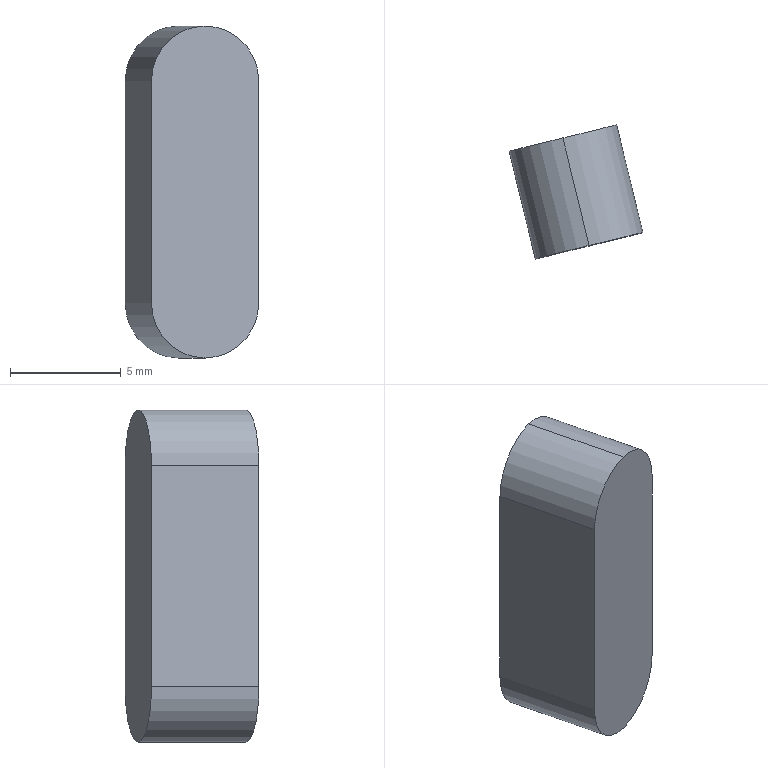Component | SolidWorks | CarrierB5-L15-1 | 1 solid | 7 faces | box 6.04 x 6.04 x 15 mm | volume 348 mm3 | plane 4 | cylinder 3 | commonest cylinder face diameters 5 x3
build123d program:
from build123d import *

# Parameters (mm, degrees)
BOSS_EXTRUDE1_DEPTH = 5


with BuildPart() as part:
    # Sketch1 → Boss-Extrude1 (new body)
    with BuildSketch(Plane(origin=(0, 0, 0), x_dir=(-1, 0, 0), z_dir=(0, 0, -1))):
        with BuildLine():
            Line((-7.5, -2.5), (2.5, -2.5))
            ThreePointArc((2.5, -2.5), (5, 0), (2.5, 2.5))
            Line((2.5, 2.5), (-7.5, 2.5))
            ThreePointArc((-7.5, 2.5), (-10, 0), (-7.5, -2.5))
        make_face()
    extrude(amount=-BOSS_EXTRUDE1_DEPTH)


solid = part.part

# Placed as in the assembly
solid = solid.moved(Location((-20.365, -8.743, 44.5), (-90, -13.725, 90)))
STEP:
#1=COLOUR_RGB('',0.7922,0.8196,0.9333);
#2=FILL_AREA_STYLE_COLOUR('',#1);
#3=FILL_AREA_STYLE('',(#2));
#4=SURFACE_STYLE_FILL_AREA(#3);
#5=SURFACE_SIDE_STYLE('',(#4));
#6=SURFACE_STYLE_USAGE(.BOTH.,#5);
#7=PRESENTATION_STYLE_ASSIGNMENT((#6));
#8=CARTESIAN_POINT('',(-0.7528,-0.1296,1.85));
#9=VERTEX_POINT('',#8);
#10=CARTESIAN_POINT('',(-0.8485,-0.153,1.949));
#11=VERTEX_POINT('',#10);
#12=CARTESIAN_POINT('',(-0.8485,-0.153,1.85));
#13=DIRECTION('',(0.2373,-0.9714,0.));
#14=DIRECTION('',(0.,0.,1.));
#15=AXIS2_PLACEMENT_3D('',#12,#13,#14);
#16=CIRCLE('',#15,0.09843);
#17=EDGE_CURVE('',#9,#11,#16,.T.);
#18=ORIENTED_EDGE('',*,*,#17,.T.);
#19=CARTESIAN_POINT('',(-0.8018,-0.3442,1.949));
#20=VERTEX_POINT('',#19);
#21=CARTESIAN_POINT('',(-0.8485,-0.153,1.949));
#22=DIRECTION('',(0.2373,-0.9714,0.));
#23=VECTOR('',#22,39.37);
#24=LINE('',#21,#23);
#25=EDGE_CURVE('',#11,#20,#24,.T.);
#26=ORIENTED_EDGE('',*,*,#25,.T.);
#27=CARTESIAN_POINT('',(-0.7061,-0.3209,1.85));
#28=VERTEX_POINT('',#27);
#29=CARTESIAN_POINT('',(-0.8018,-0.3442,1.85));
#30=DIRECTION('',(0.2373,-0.9714,0.));
#31=DIRECTION('',(0.,0.,1.));
#32=AXIS2_PLACEMENT_3D('',#29,#30,#31);
#33=CIRCLE('',#32,0.09843);
#34=EDGE_CURVE('',#28,#20,#33,.T.);
#35=ORIENTED_EDGE('',*,*,#34,.F.);
#36=CARTESIAN_POINT('',(-0.7528,-0.1296,1.85));
#37=DIRECTION('',(0.2373,-0.9714,0.));
#38=VECTOR('',#37,39.37);
#39=LINE('',#36,#38);
#40=EDGE_CURVE('',#9,#28,#39,.T.);
#41=ORIENTED_EDGE('',*,*,#40,.F.);
#42=EDGE_LOOP('',(#18,#26,#35,#41));
#43=FACE_OUTER_BOUND('',#42,.T.);
#44=CARTESIAN_POINT('',(-0.8485,-0.153,1.85));
#45=DIRECTION('',(0.2373,-0.9714,0.));
#46=DIRECTION('',(0.,0.,1.));
#47=AXIS2_PLACEMENT_3D('',#44,#45,#46);
#48=CYLINDRICAL_SURFACE('',#47,0.09843);
#49=ADVANCED_FACE('',(#43),#48,.T.);
#50=CARTESIAN_POINT('',(-0.8974,-0.3676,1.457));
#51=VERTEX_POINT('',#50);
#52=CARTESIAN_POINT('',(-0.7061,-0.3209,1.457));
#53=VERTEX_POINT('',#52);
#54=CARTESIAN_POINT('',(-0.8018,-0.3442,1.457));
#55=DIRECTION('',(0.2373,-0.9714,0.));
#56=DIRECTION('',(0.,0.,1.));
#57=AXIS2_PLACEMENT_3D('',#54,#55,#56);
#58=CIRCLE('',#57,0.09843);
#59=EDGE_CURVE('',#51,#53,#58,.T.);
#60=ORIENTED_EDGE('',*,*,#59,.F.);
#61=CARTESIAN_POINT('',(-0.9441,-0.1763,1.457));
#62=VERTEX_POINT('',#61);
#63=CARTESIAN_POINT('',(-0.9441,-0.1763,1.457));
#64=DIRECTION('',(0.2373,-0.9714,0.));
#65=VECTOR('',#64,39.37);
#66=LINE('',#63,#65);
#67=EDGE_CURVE('',#62,#51,#66,.T.);
#68=ORIENTED_EDGE('',*,*,#67,.F.);
#69=CARTESIAN_POINT('',(-0.7528,-0.1296,1.457));
#70=VERTEX_POINT('',#69);
#71=CARTESIAN_POINT('',(-0.8485,-0.153,1.457));
#72=DIRECTION('',(0.2373,-0.9714,0.));
#73=DIRECTION('',(0.,0.,1.));
#74=AXIS2_PLACEMENT_3D('',#71,#72,#73);
#75=CIRCLE('',#74,0.09843);
#76=EDGE_CURVE('',#62,#70,#75,.T.);
#77=ORIENTED_EDGE('',*,*,#76,.T.);
#78=CARTESIAN_POINT('',(-0.7528,-0.1296,1.457));
#79=DIRECTION('',(0.2373,-0.9714,0.));
#80=VECTOR('',#79,39.37);
#81=LINE('',#78,#80);
#82=EDGE_CURVE('',#70,#53,#81,.T.);
#83=ORIENTED_EDGE('',*,*,#82,.T.);
#84=EDGE_LOOP('',(#60,#68,#77,#83));
#85=FACE_OUTER_BOUND('',#84,.T.);
#86=CARTESIAN_POINT('',(-0.8485,-0.153,1.457));
#87=DIRECTION('',(0.2373,-0.9714,0.));
#88=DIRECTION('',(0.,0.,1.));
#89=AXIS2_PLACEMENT_3D('',#86,#87,#88);
#90=CYLINDRICAL_SURFACE('',#89,0.09843);
#91=ADVANCED_FACE('',(#85),#90,.T.);
#92=CARTESIAN_POINT('',(-0.8974,-0.3676,1.85));
#93=VERTEX_POINT('',#92);
#94=CARTESIAN_POINT('',(-0.8974,-0.3676,1.85));
#95=DIRECTION('',(0.,0.,-1.));
#96=VECTOR('',#95,39.37);
#97=LINE('',#94,#96);
#98=EDGE_CURVE('',#93,#51,#97,.T.);
#99=ORIENTED_EDGE('',*,*,#98,.F.);
#100=CARTESIAN_POINT('',(-0.9441,-0.1763,1.85));
#101=VERTEX_POINT('',#100);
#102=CARTESIAN_POINT('',(-0.9441,-0.1763,1.85));
#103=DIRECTION('',(0.2373,-0.9714,0.));
#104=VECTOR('',#103,39.37);
#105=LINE('',#102,#104);
#106=EDGE_CURVE('',#101,#93,#105,.T.);
#107=ORIENTED_EDGE('',*,*,#106,.F.);
#108=CARTESIAN_POINT('',(-0.9441,-0.1763,1.85));
#109=DIRECTION('',(0.,0.,-1.));
#110=VECTOR('',#109,39.37);
#111=LINE('',#108,#110);
#112=EDGE_CURVE('',#101,#62,#111,.T.);
#113=ORIENTED_EDGE('',*,*,#112,.T.);
#114=ORIENTED_EDGE('',*,*,#67,.T.);
#115=EDGE_LOOP('',(#99,#107,#113,#114));
#116=FACE_OUTER_BOUND('',#115,.T.);
#117=CARTESIAN_POINT('',(-0.9441,-0.1763,1.85));
#118=DIRECTION('',(-0.9714,-0.2373,-0.));
#119=DIRECTION('',(-0.,-0.,1.));
#120=AXIS2_PLACEMENT_3D('',#117,#118,#119);
#121=PLANE('',#120);
#122=ADVANCED_FACE('',(#116),#121,.T.);
#123=ORIENTED_EDGE('',*,*,#25,.F.);
#124=CARTESIAN_POINT('',(-0.8485,-0.153,1.85));
#125=DIRECTION('',(0.2373,-0.9714,0.));
#126=DIRECTION('',(0.,0.,1.));
#127=AXIS2_PLACEMENT_3D('',#124,#125,#126);
#128=CIRCLE('',#127,0.09843);
#129=EDGE_CURVE('',#11,#101,#128,.T.);
#130=ORIENTED_EDGE('',*,*,#129,.T.);
#131=ORIENTED_EDGE('',*,*,#106,.T.);
#132=CARTESIAN_POINT('',(-0.8018,-0.3442,1.85));
#133=DIRECTION('',(0.2373,-0.9714,0.));
#134=DIRECTION('',(0.,0.,1.));
#135=AXIS2_PLACEMENT_3D('',#132,#133,#134);
#136=CIRCLE('',#135,0.09843);
#137=EDGE_CURVE('',#20,#93,#136,.T.);
#138=ORIENTED_EDGE('',*,*,#137,.F.);
#139=EDGE_LOOP('',(#123,#130,#131,#138));
#140=FACE_OUTER_BOUND('',#139,.T.);
#141=CARTESIAN_POINT('',(-0.8485,-0.153,1.85));
#142=DIRECTION('',(0.2373,-0.9714,0.));
#143=DIRECTION('',(0.,0.,1.));
#144=AXIS2_PLACEMENT_3D('',#141,#142,#143);
#145=CYLINDRICAL_SURFACE('',#144,0.09843);
#146=ADVANCED_FACE('',(#140),#145,.T.);
#147=CARTESIAN_POINT('',(-0.7061,-0.3209,1.457));
#148=DIRECTION('',(0.,0.,1.));
#149=VECTOR('',#148,39.37);
#150=LINE('',#147,#149);
#151=EDGE_CURVE('',#53,#28,#150,.T.);
#152=ORIENTED_EDGE('',*,*,#151,.F.);
#153=ORIENTED_EDGE('',*,*,#82,.F.);
#154=CARTESIAN_POINT('',(-0.7528,-0.1296,1.457));
#155=DIRECTION('',(0.,0.,1.));
#156=VECTOR('',#155,39.37);
#157=LINE('',#154,#156);
#158=EDGE_CURVE('',#70,#9,#157,.T.);
#159=ORIENTED_EDGE('',*,*,#158,.T.);
#160=ORIENTED_EDGE('',*,*,#40,.T.);
#161=EDGE_LOOP('',(#152,#153,#159,#160));
#162=FACE_OUTER_BOUND('',#161,.T.);
#163=CARTESIAN_POINT('',(-0.7528,-0.1296,1.457));
#164=DIRECTION('',(0.9714,0.2373,0.));
#165=DIRECTION('',(0.2373,-0.9714,0.));
#166=AXIS2_PLACEMENT_3D('',#163,#164,#165);
#167=PLANE('',#166);
#168=ADVANCED_FACE('',(#162),#167,.T.);
#169=ORIENTED_EDGE('',*,*,#76,.F.);
#170=ORIENTED_EDGE('',*,*,#112,.F.);
#171=ORIENTED_EDGE('',*,*,#129,.F.);
#172=ORIENTED_EDGE('',*,*,#17,.F.);
#173=ORIENTED_EDGE('',*,*,#158,.F.);
#174=EDGE_LOOP('',(#169,#170,#171,#172,#173));
#175=FACE_OUTER_BOUND('',#174,.T.);
#176=CARTESIAN_POINT('',(-0.8485,-0.153,1.457));
#177=DIRECTION('',(0.2373,-0.9714,0.));
#178=DIRECTION('',(0.,0.,1.));
#179=AXIS2_PLACEMENT_3D('',#176,#177,#178);
#180=PLANE('',#179);
#181=ADVANCED_FACE('',(#175),#180,.F.);
#182=ORIENTED_EDGE('',*,*,#59,.T.);
#183=ORIENTED_EDGE('',*,*,#151,.T.);
#184=ORIENTED_EDGE('',*,*,#34,.T.);
#185=ORIENTED_EDGE('',*,*,#137,.T.);
#186=ORIENTED_EDGE('',*,*,#98,.T.);
#187=EDGE_LOOP('',(#182,#183,#184,#185,#186));
#188=FACE_OUTER_BOUND('',#187,.T.);
#189=CARTESIAN_POINT('',(-0.8018,-0.3442,1.457));
#190=DIRECTION('',(0.2373,-0.9714,0.));
#191=DIRECTION('',(0.,0.,1.));
#192=AXIS2_PLACEMENT_3D('',#189,#190,#191);
#193=PLANE('',#192);
#194=ADVANCED_FACE('',(#188),#193,.T.);
#195=CLOSED_SHELL('',(#49,#91,#122,#146,#168,#181,#194));
#196=MANIFOLD_SOLID_BREP('',#195);
#197=STYLED_ITEM('',(#7),#196);
#198=(LENGTH_UNIT()NAMED_UNIT(*)SI_UNIT($,.METRE.));
#199=LENGTH_MEASURE_WITH_UNIT(LENGTH_MEASURE(0.0254),#198);
#200=DIMENSIONAL_EXPONENTS(1.,0.,0.,0.,0.,0.,0.);
#201=(CONVERSION_BASED_UNIT('',#199)LENGTH_UNIT()NAMED_UNIT(#200));
#202=UNCERTAINTY_MEASURE_WITH_UNIT(LENGTH_MEASURE(0.00001),#201,'','');
#203=(NAMED_UNIT(*)PLANE_ANGLE_UNIT()SI_UNIT($,.RADIAN.));
#204=(NAMED_UNIT(*)SI_UNIT($,.STERADIAN.)SOLID_ANGLE_UNIT());
#205=(GEOMETRIC_REPRESENTATION_CONTEXT(3)GLOBAL_UNCERTAINTY_ASSIGNED_CONTEXT((#202))GLOBAL_UNIT_ASSIGNED_CONTEXT((#201,#203,#204))REPRESENTATION_CONTEXT('',''));
#206=MECHANICAL_DESIGN_GEOMETRIC_PRESENTATION_REPRESENTATION('',(#197),#205);
#207=PRESENTATION_LAYER_ASSIGNMENT('','',(#197));
#208=CARTESIAN_POINT('',(0.,0.,0.));
#209=DIRECTION('',(0.,0.,1.));
#210=DIRECTION('',(1.,0.,0.));
#211=AXIS2_PLACEMENT_3D('',#208,#209,#210);
#212=(LENGTH_UNIT()NAMED_UNIT(*)SI_UNIT($,.METRE.));
#213=LENGTH_MEASURE_WITH_UNIT(LENGTH_MEASURE(0.0254),#212);
#214=DIMENSIONAL_EXPONENTS(1.,0.,0.,0.,0.,0.,0.);
#215=(CONVERSION_BASED_UNIT('',#213)LENGTH_UNIT()NAMED_UNIT(#214));
#216=UNCERTAINTY_MEASURE_WITH_UNIT(LENGTH_MEASURE(0.00001),#215,'','');
#217=(NAMED_UNIT(*)PLANE_ANGLE_UNIT()SI_UNIT($,.RADIAN.));
#218=(NAMED_UNIT(*)SI_UNIT($,.STERADIAN.)SOLID_ANGLE_UNIT());
#219=(GEOMETRIC_REPRESENTATION_CONTEXT(3)GLOBAL_UNCERTAINTY_ASSIGNED_CONTEXT((#216))GLOBAL_UNIT_ASSIGNED_CONTEXT((#215,#217,#218))REPRESENTATION_CONTEXT('',''));
#220=ADVANCED_BREP_SHAPE_REPRESENTATION('',(#196,#211),#219);